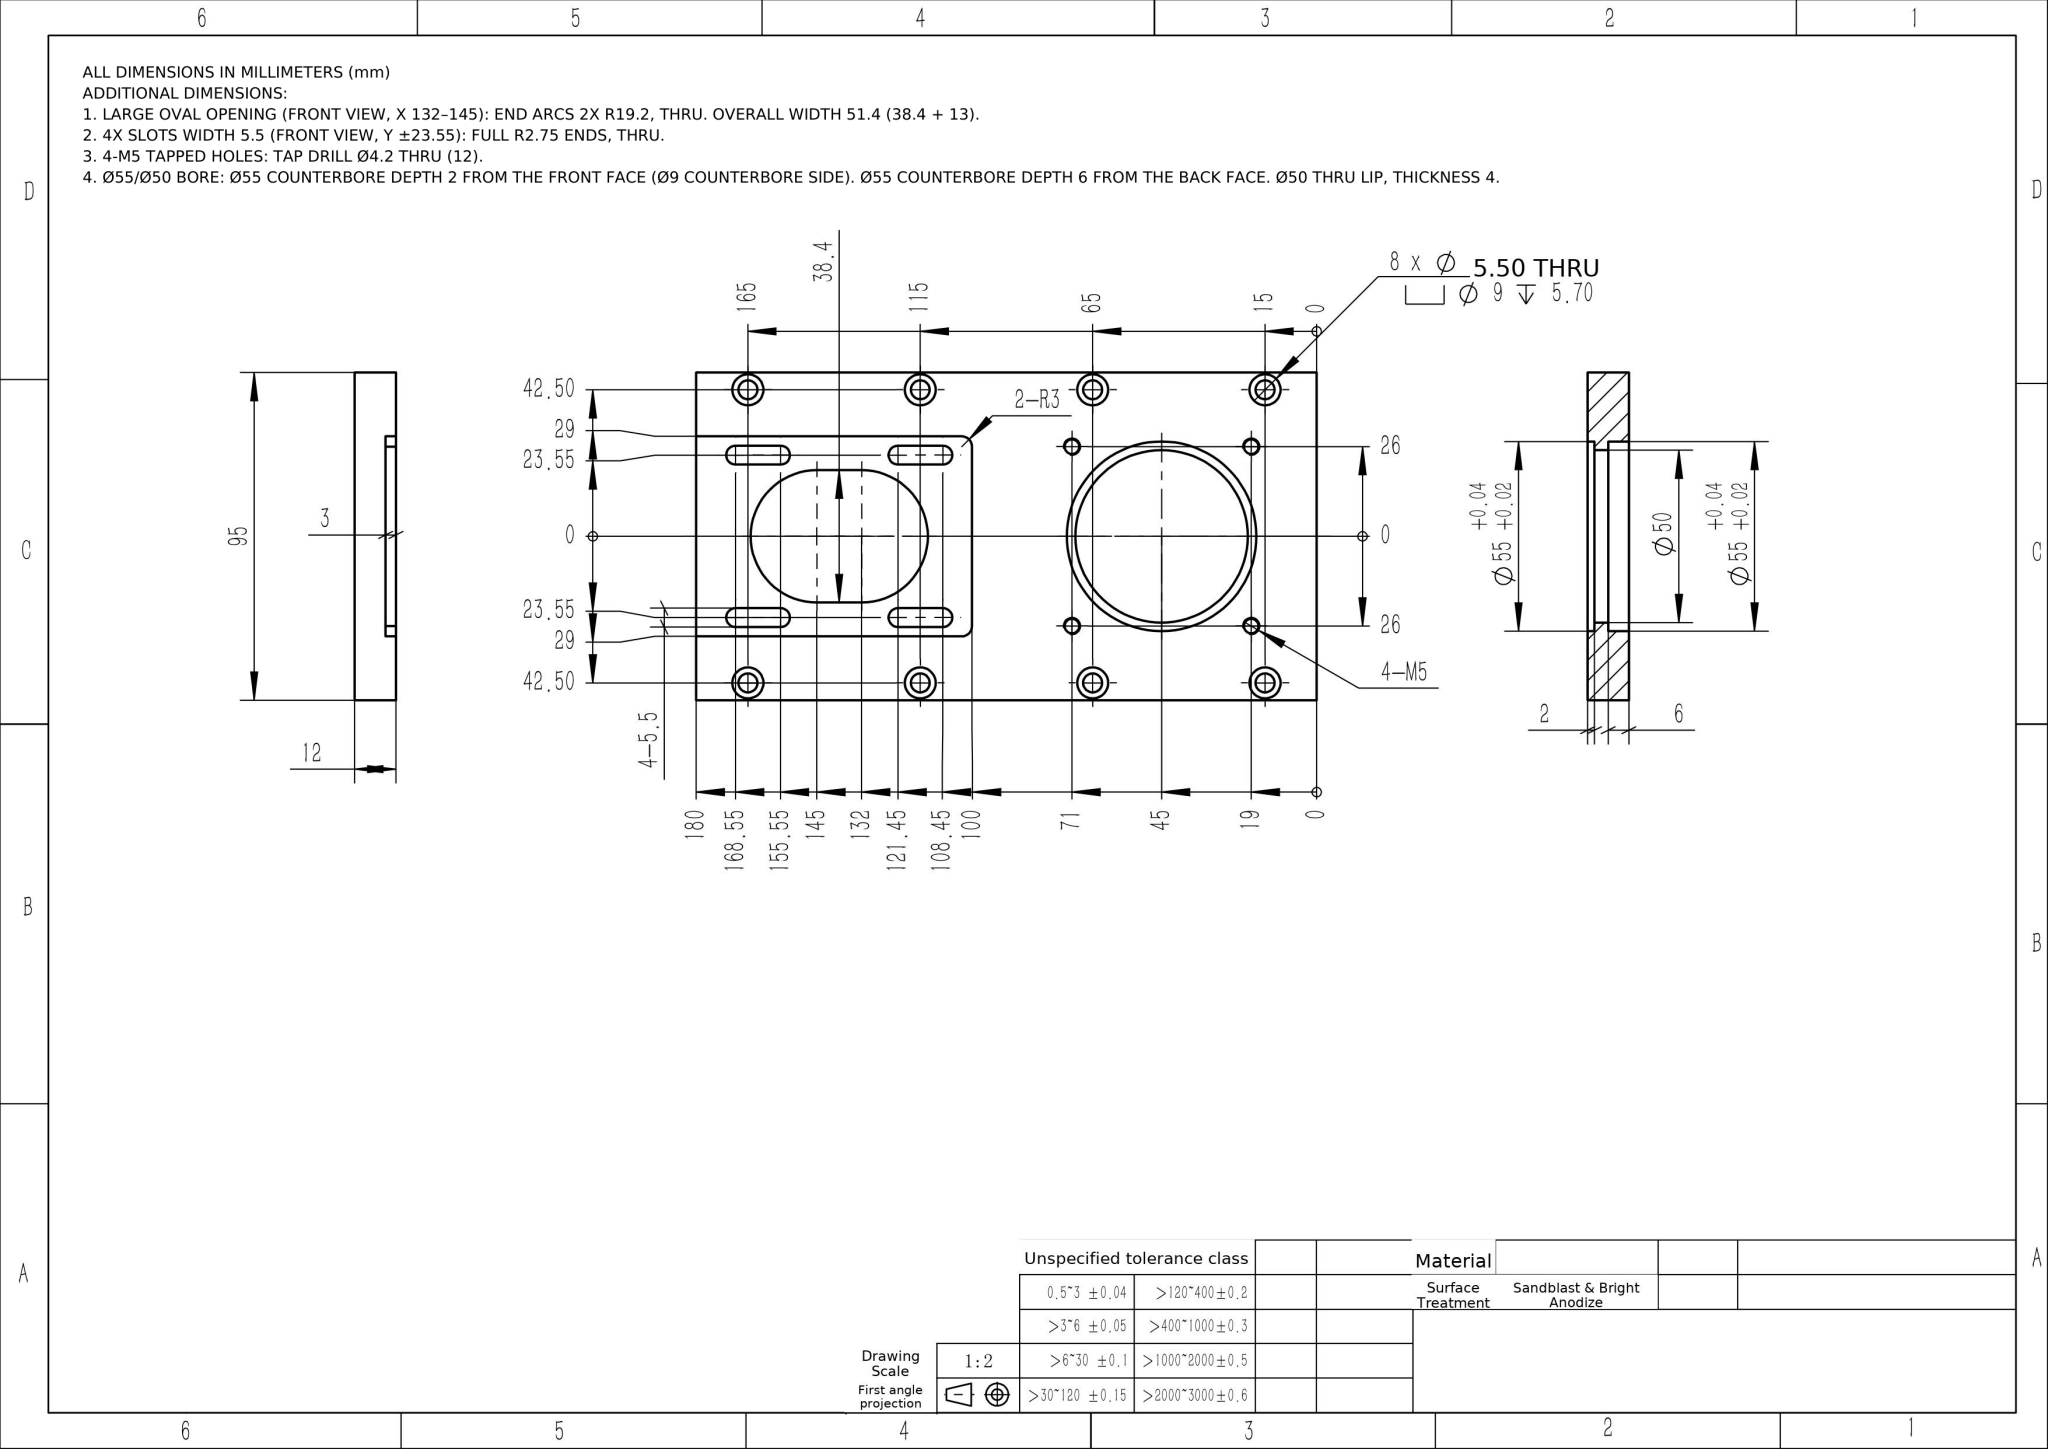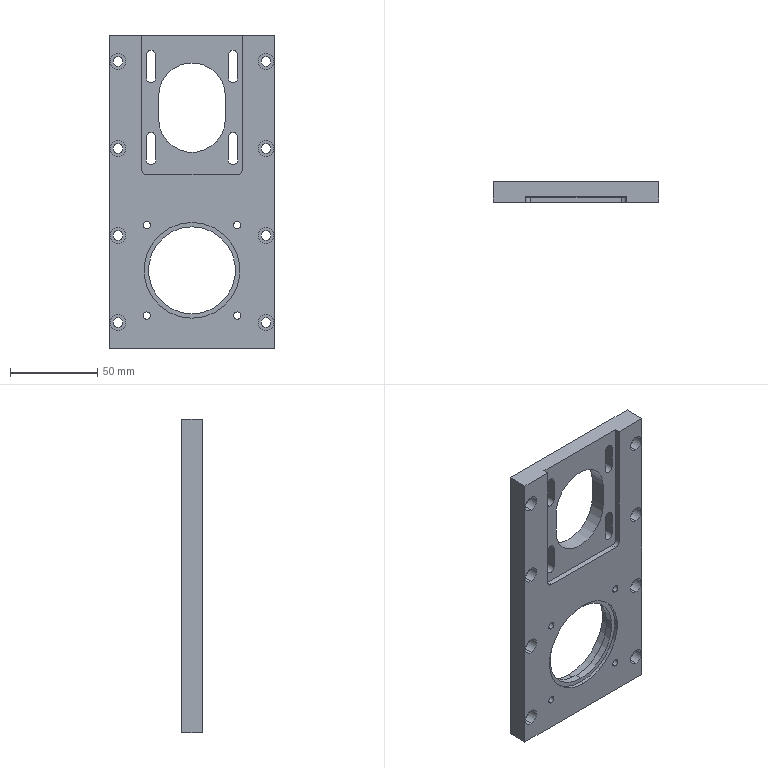Part | NX | mm | 1 solid | 92 faces | box 95 x 12 x 180 mm | volume 141322 mm3 | cylinder 62 | plane 30 | commonest cylinder face diameters 5.5 x28 9 x16 4.2 x8 55 x4 50 x2 6 x2 38.4 x2